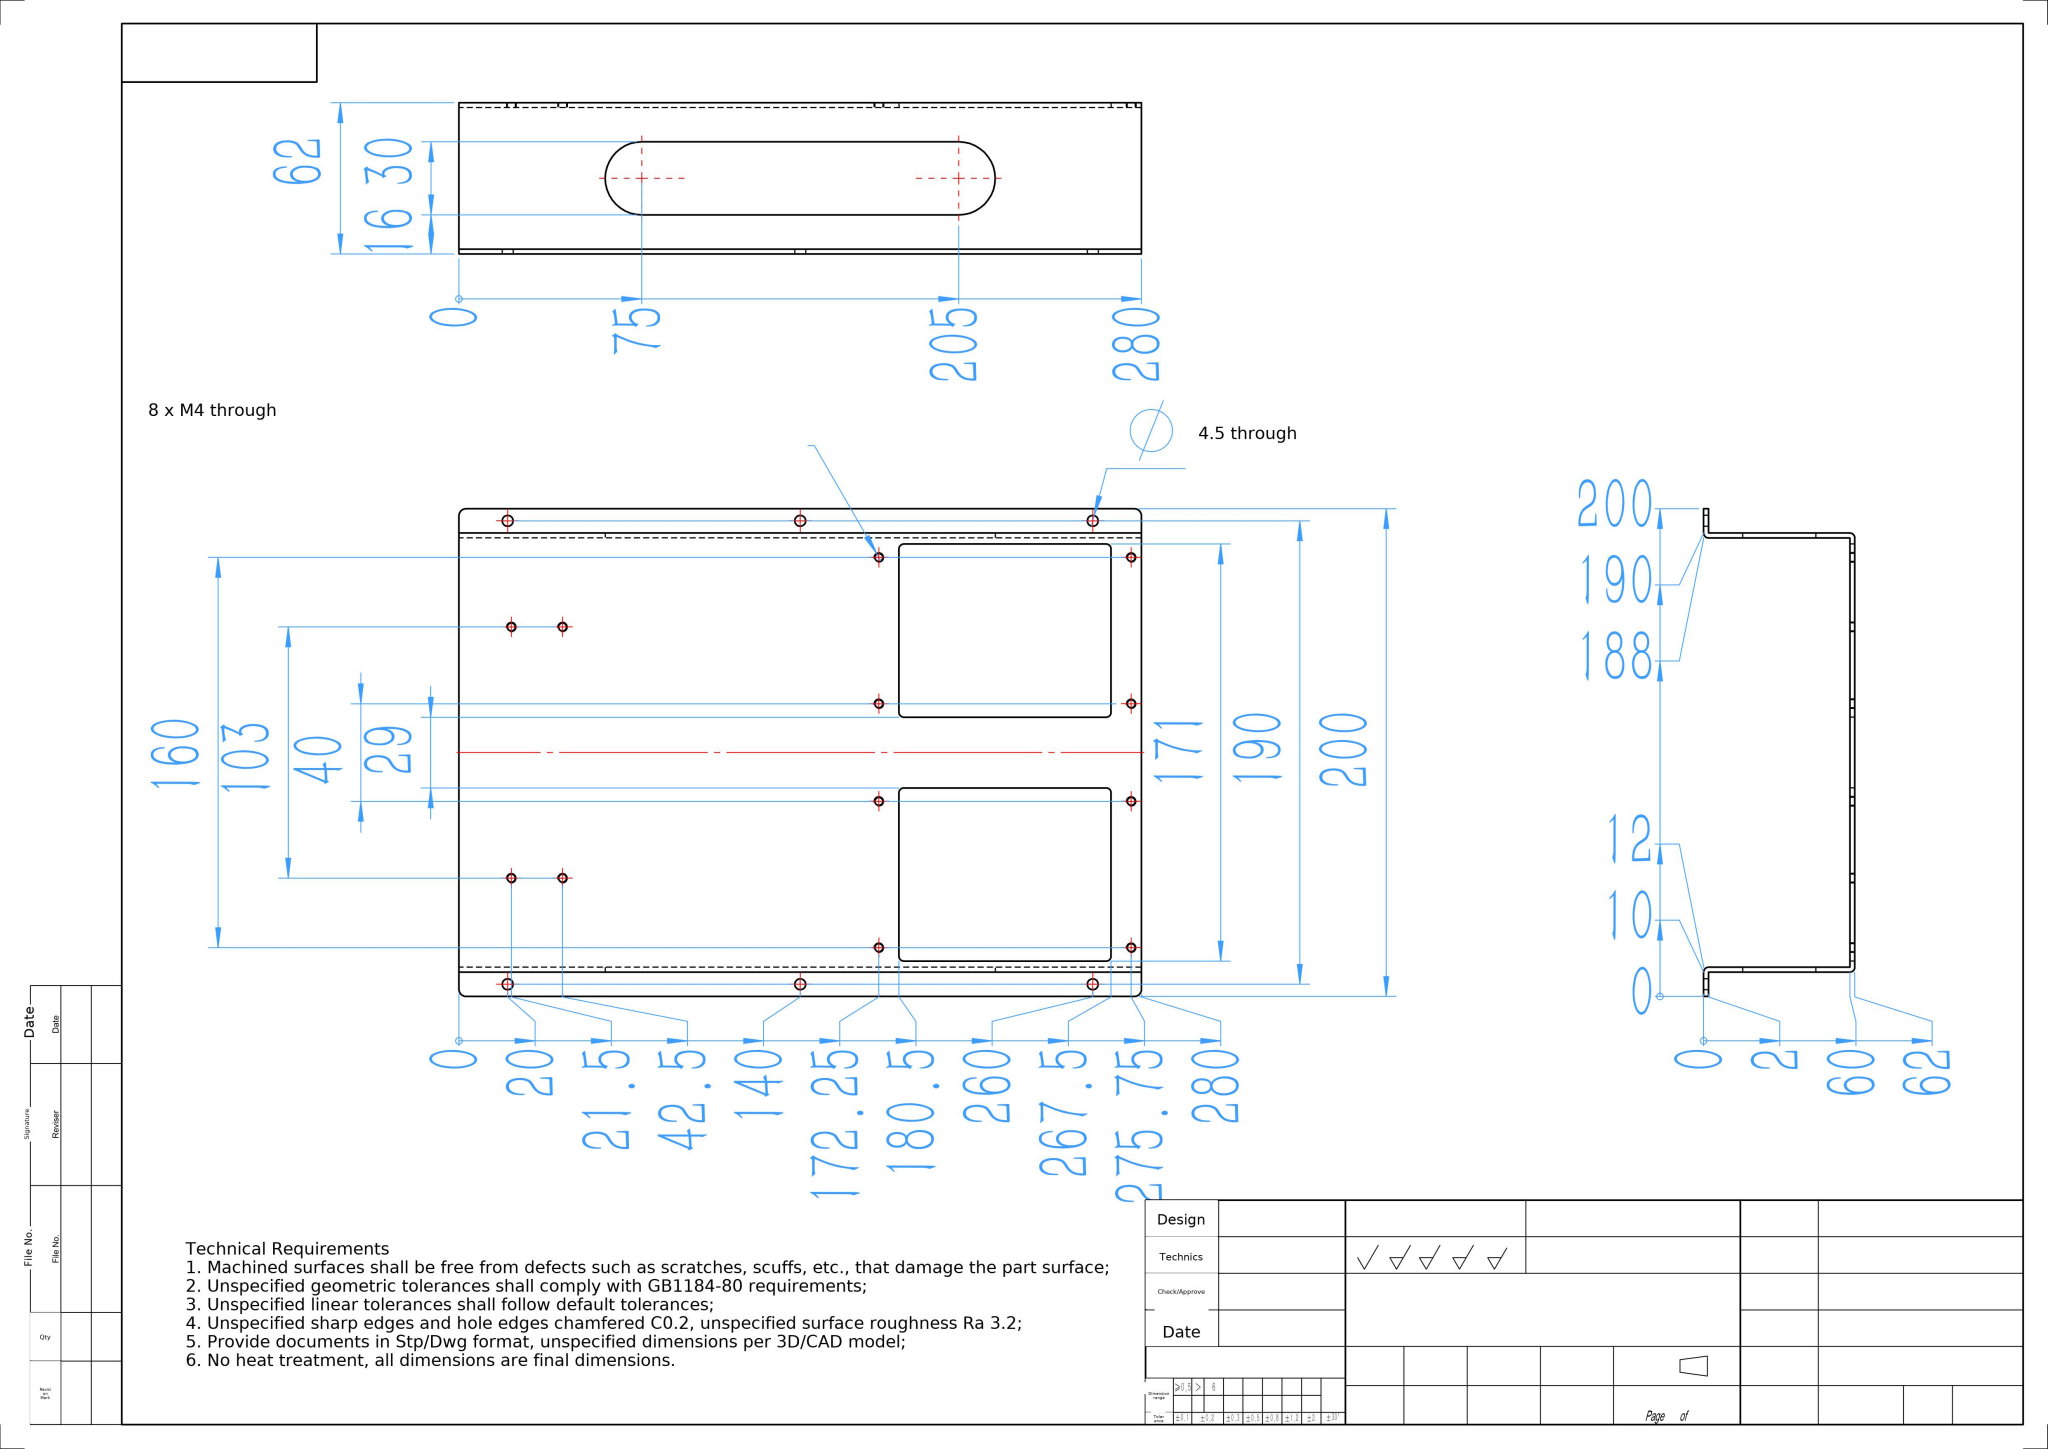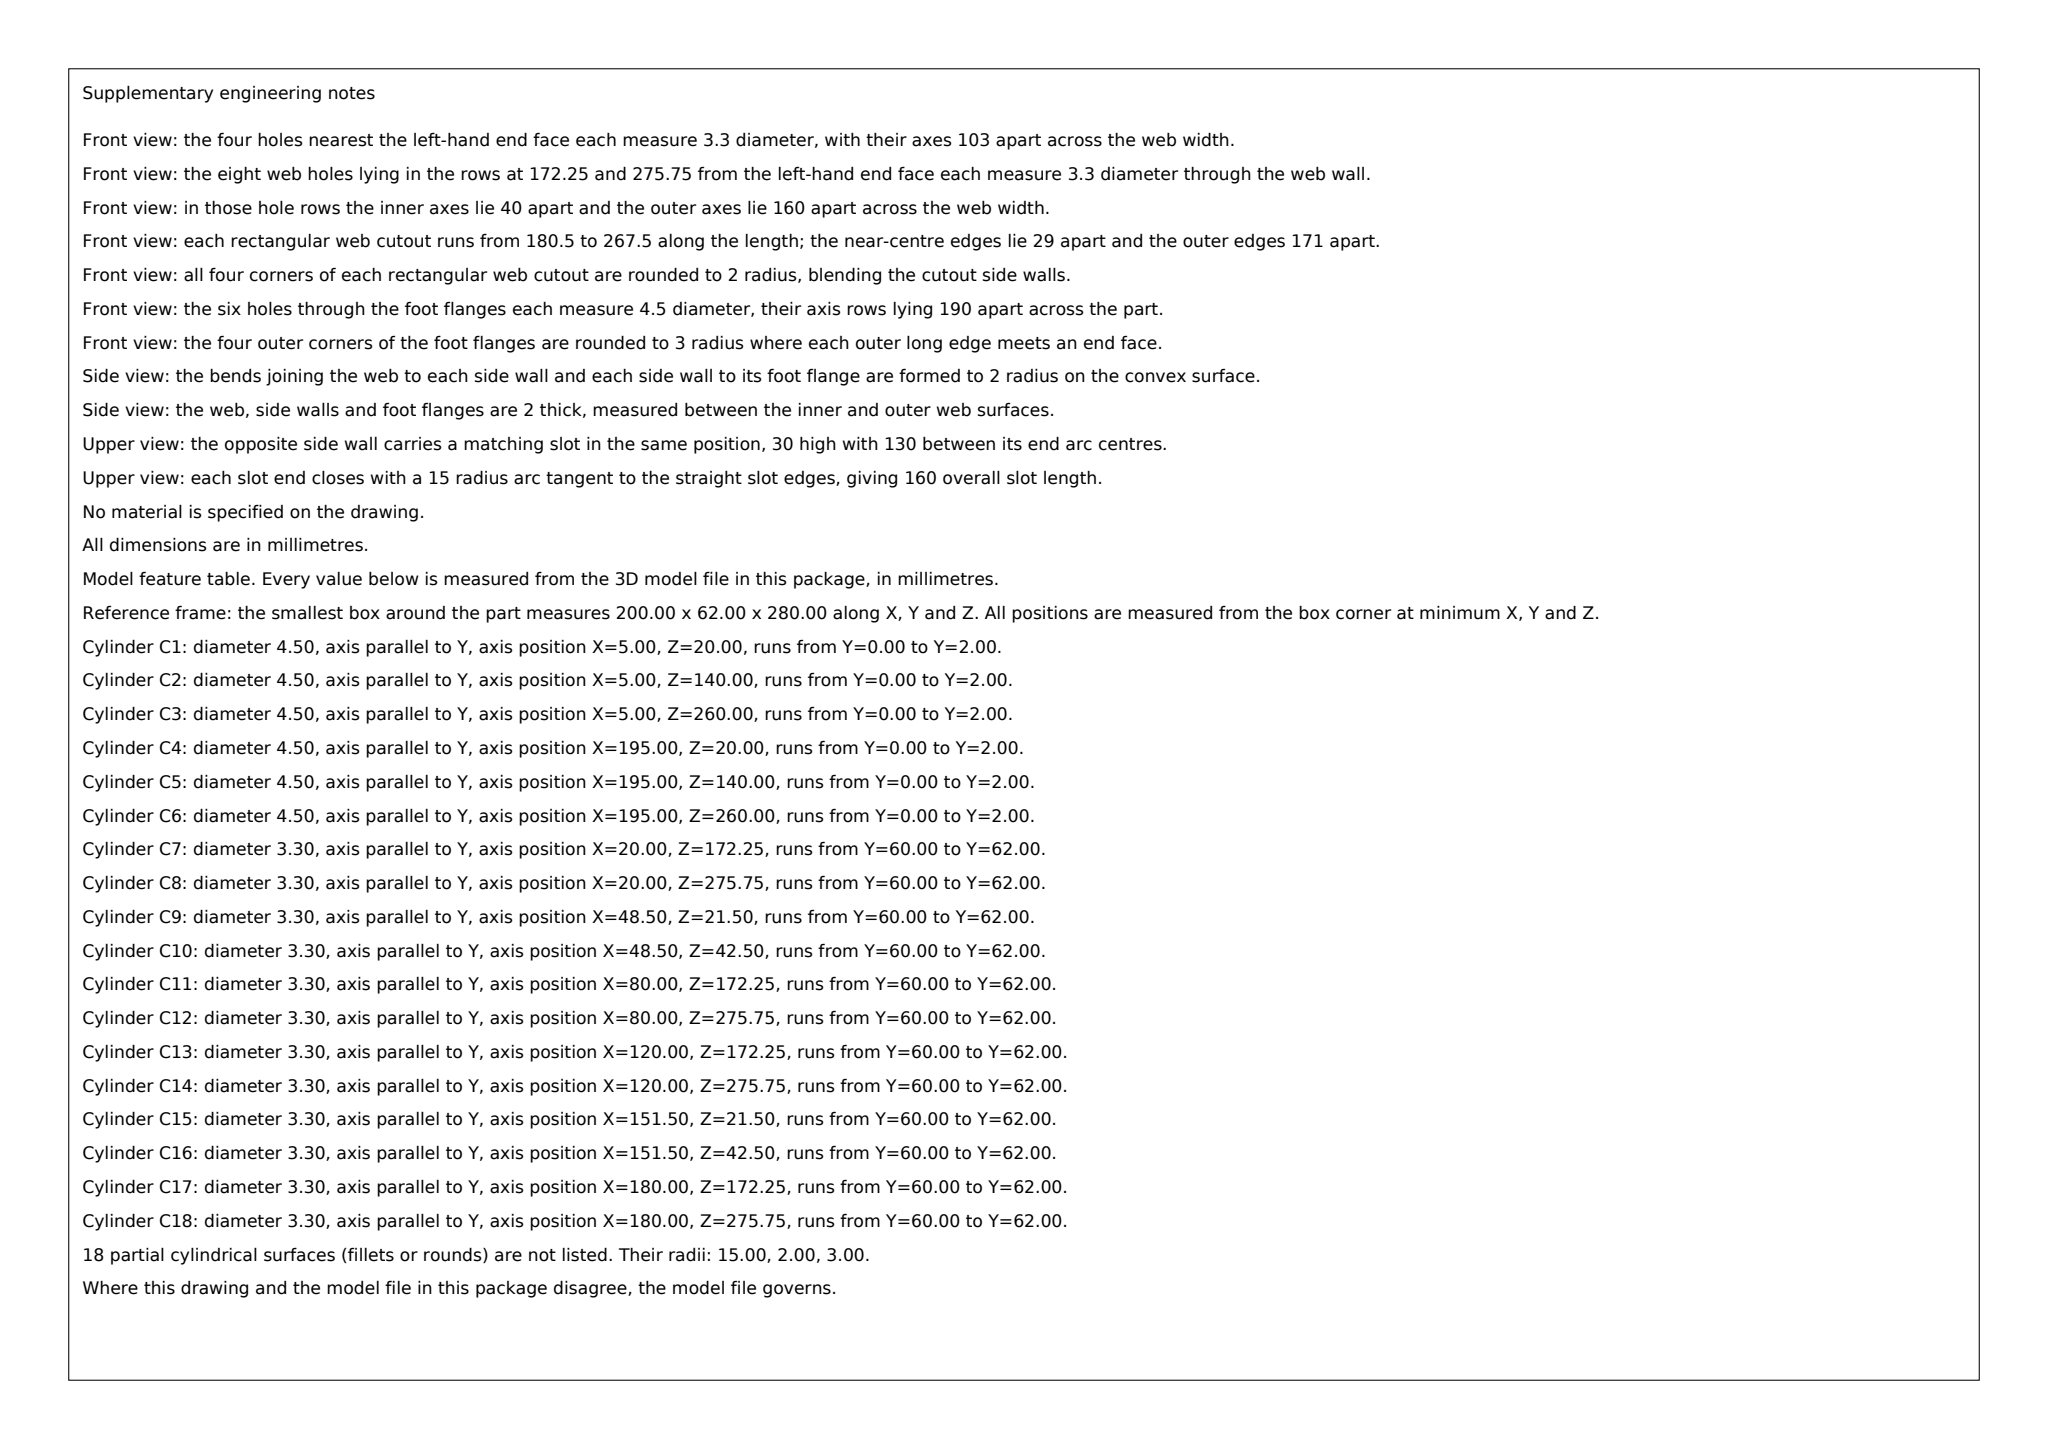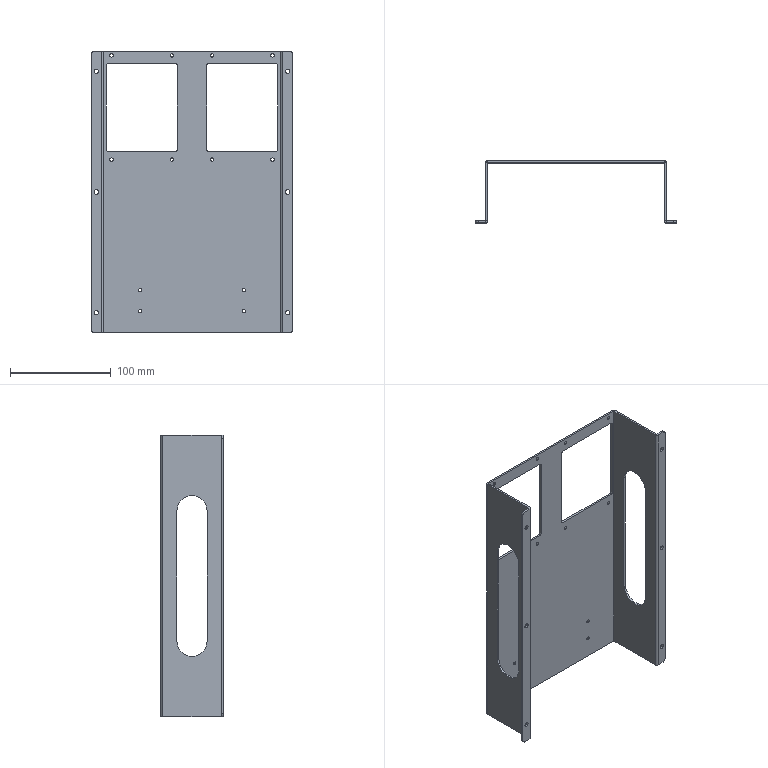Part | SolidWorks | mm | 1 solid | 98 faces | box 200 x 62 x 280 mm | volume 134705 mm3 | cylinder 56 | plane 42 | commonest cylinder face diameters 3.3 x24 4.5 x12 4 x12 30 x4 6 x4
Drawing notes:
2X CUTOUT THRU 71 x 87, 8X R2; X 14.5-85.5 & 114.5-185.5, Z 180.5-267.5 | from the solid: x planes 14.5/85.5 & 114.5/185.5 (71 wide); z planes 180.5/267.5 (87); 8X R2 corners
4X Ø3.3 THRU 2 THK FLG AT X 48.5 & 151.5, Z 21.5 & 42.5 | from the solid: Ø3.3 y-axis holes, len 2.0, at x=48.5/151.5, z=21.5 & 42.5
8X M4 THRU AT X 16.5, 83.5, 116.5, 183.5; Z 182.5 & 265.5 | from the solid: Ø4.0 y-axis holes at x=16.5/83.5/116.5/183.5, z=182.5 & 265.5
4X Ø3.3 THRU 2 THK FLG AT X 48.5 & 151.5, Z 21.5 & 42.5 (from bbox min corner) | from the solid: cylinders dia 3.3 axis y at [48.5,-,21.5], [48.5,-,42.5], [151.5,-,21.5], [151.5,-,42.5], length 2.0
8X Ø3.3 THRU 2 THK FLG AT X 20, 80, 120 & 180; Z 172.25 & 275.75 (from bbox min corner) | from the solid: cylinders dia 3.3 axis y at Z 172.25 and Z 275.75, X 20/80/120/180, length 2.0
2X (BOTH FLANGES) SLOT 30 WIDE, R15 ENDS, THRU; SLOT END CENTERS AT Z 75 & 205, Y 31 FROM BOTTOM (Y 16 TO 46) | from the solid: cylinders dia 30.0 axis x at [-,31.0,75.0] and [-,31.0,205.0], each count 2; y planes 16.0 and 46.0 each count 2
8X Ø3.3 THRU 2 THK FLANGE AT X 20, 80, 120 & 180; Z 172.25 & 275.75 (from bbox min corner) | from the solid: cylinders dia 3.3, axis y, length 2.0 at [20,172.25],[80,172.25],[120,172.25],[180,172.25],[20,275.75],[80,275.75],[120,275.75],[180,275.75]
4X Ø3.3 THRU 2 THK FLANGE AT X 48.5 & 151.5; Z 21.5 & 42.5 (replaces garbled callout) | from the solid: cylinders dia 3.3, axis y, length 2.0 at [48.5,21.5],[48.5,42.5],[151.5,21.5],[151.5,42.5]
2X SLOT 30 WIDE WITH R15 ENDS, THRU 2 THK FLANGE, BOTH FLANGES (Y 16-46); END CENTERS AT Z 75 & 205 | from the solid: cylinders dia 30, axis x, length 2.0 at z=75 and z=205 each count 2 (one per flange); y planes 16.0 and 46.0 each count 2
4X Ø3.3 THRU 2 THK FLANGE AT X 48.5 & 151.5, Z 21.5 & 42.5 (FROM BBOX MIN CORNER) | from the solid: cylinders dia 3.3 axis y at [48.5,null,21.5], [48.5,null,42.5], [151.5,null,21.5], [151.5,null,42.5], length 2.0
8X Ø3.3 THRU 2 THK FLANGE AT X 20, 80, 120 & 180; Z 172.25 & 275.75 (FROM BBOX MIN CORNER) | from the solid: cylinders dia 3.3 axis y at [20/80/120/180,null,172.25] and [20/80/120/180,null,275.75], length 2.0
2X SLOT 30 WIDE, R15 ENDS, THRU 2 THK FLANGE - BOTH FLANGES (Y 16 TO 46); SLOT END CENTERS AT Z 75 & 205, Y 31 FROM BOTTOM | from the solid: cylinders dia 30.0 axis x at [null,31.0,75.0] count 2 and [null,31.0,205.0] count 2, length 2.0; y planes at 16.0 and 46.0 count 2 each
4X Ø6 THRU 2 THK END LIP AT X 3 & 197, Z 3 & 277 (FROM BBOX MIN CORNER) | from the solid: cylinders dia 6.0 axis y, length 2, at (x,z) = (3,3), (3,277), (197,3), (197,277)
6X Ø4.5 THRU 2 THK FLANGE AT X 5 & 195; Z 20, 140 & 260 (FROM BBOX MIN CORNER) | from the solid: cylinders dia 4.5 axis y, length 2, at (x,z) = (5,20),(5,140),(5,260),(195,20),(195,140),(195,260)
4X Ø3.3 THRU 2 THK FLANGE AT X 48.5 & 151.5; Z 21.5 & 42.5 (FROM BBOX MIN CORNER) | from the solid: cylinders dia 3.3 axis y, length 2, at (x,z) = (48.5,21.5),(48.5,42.5),(151.5,21.5),(151.5,42.5)